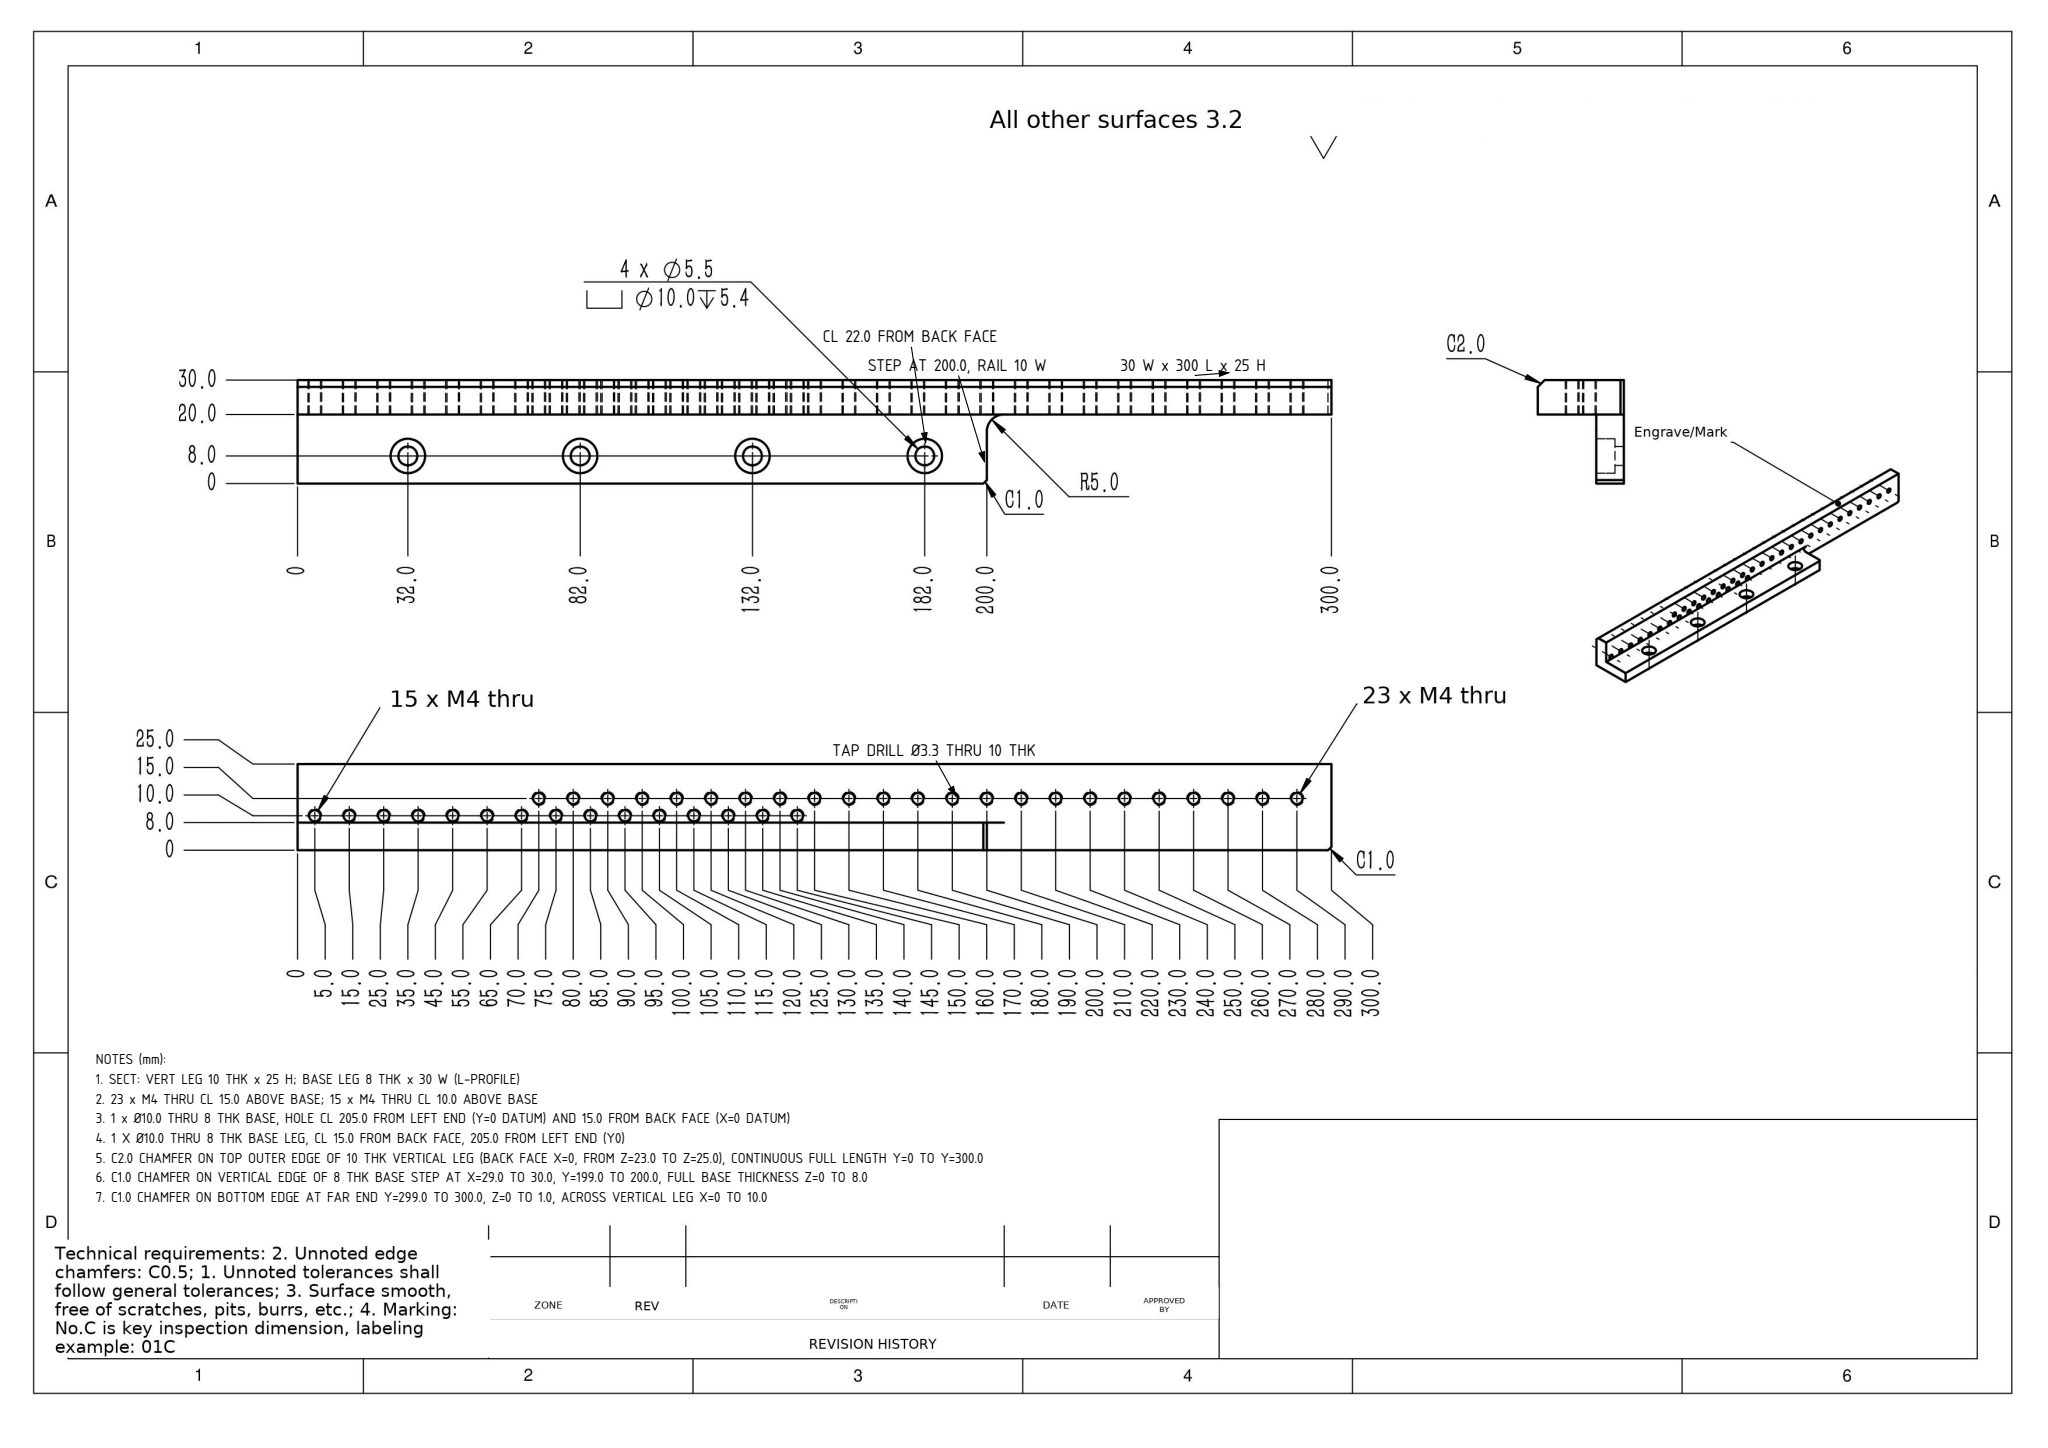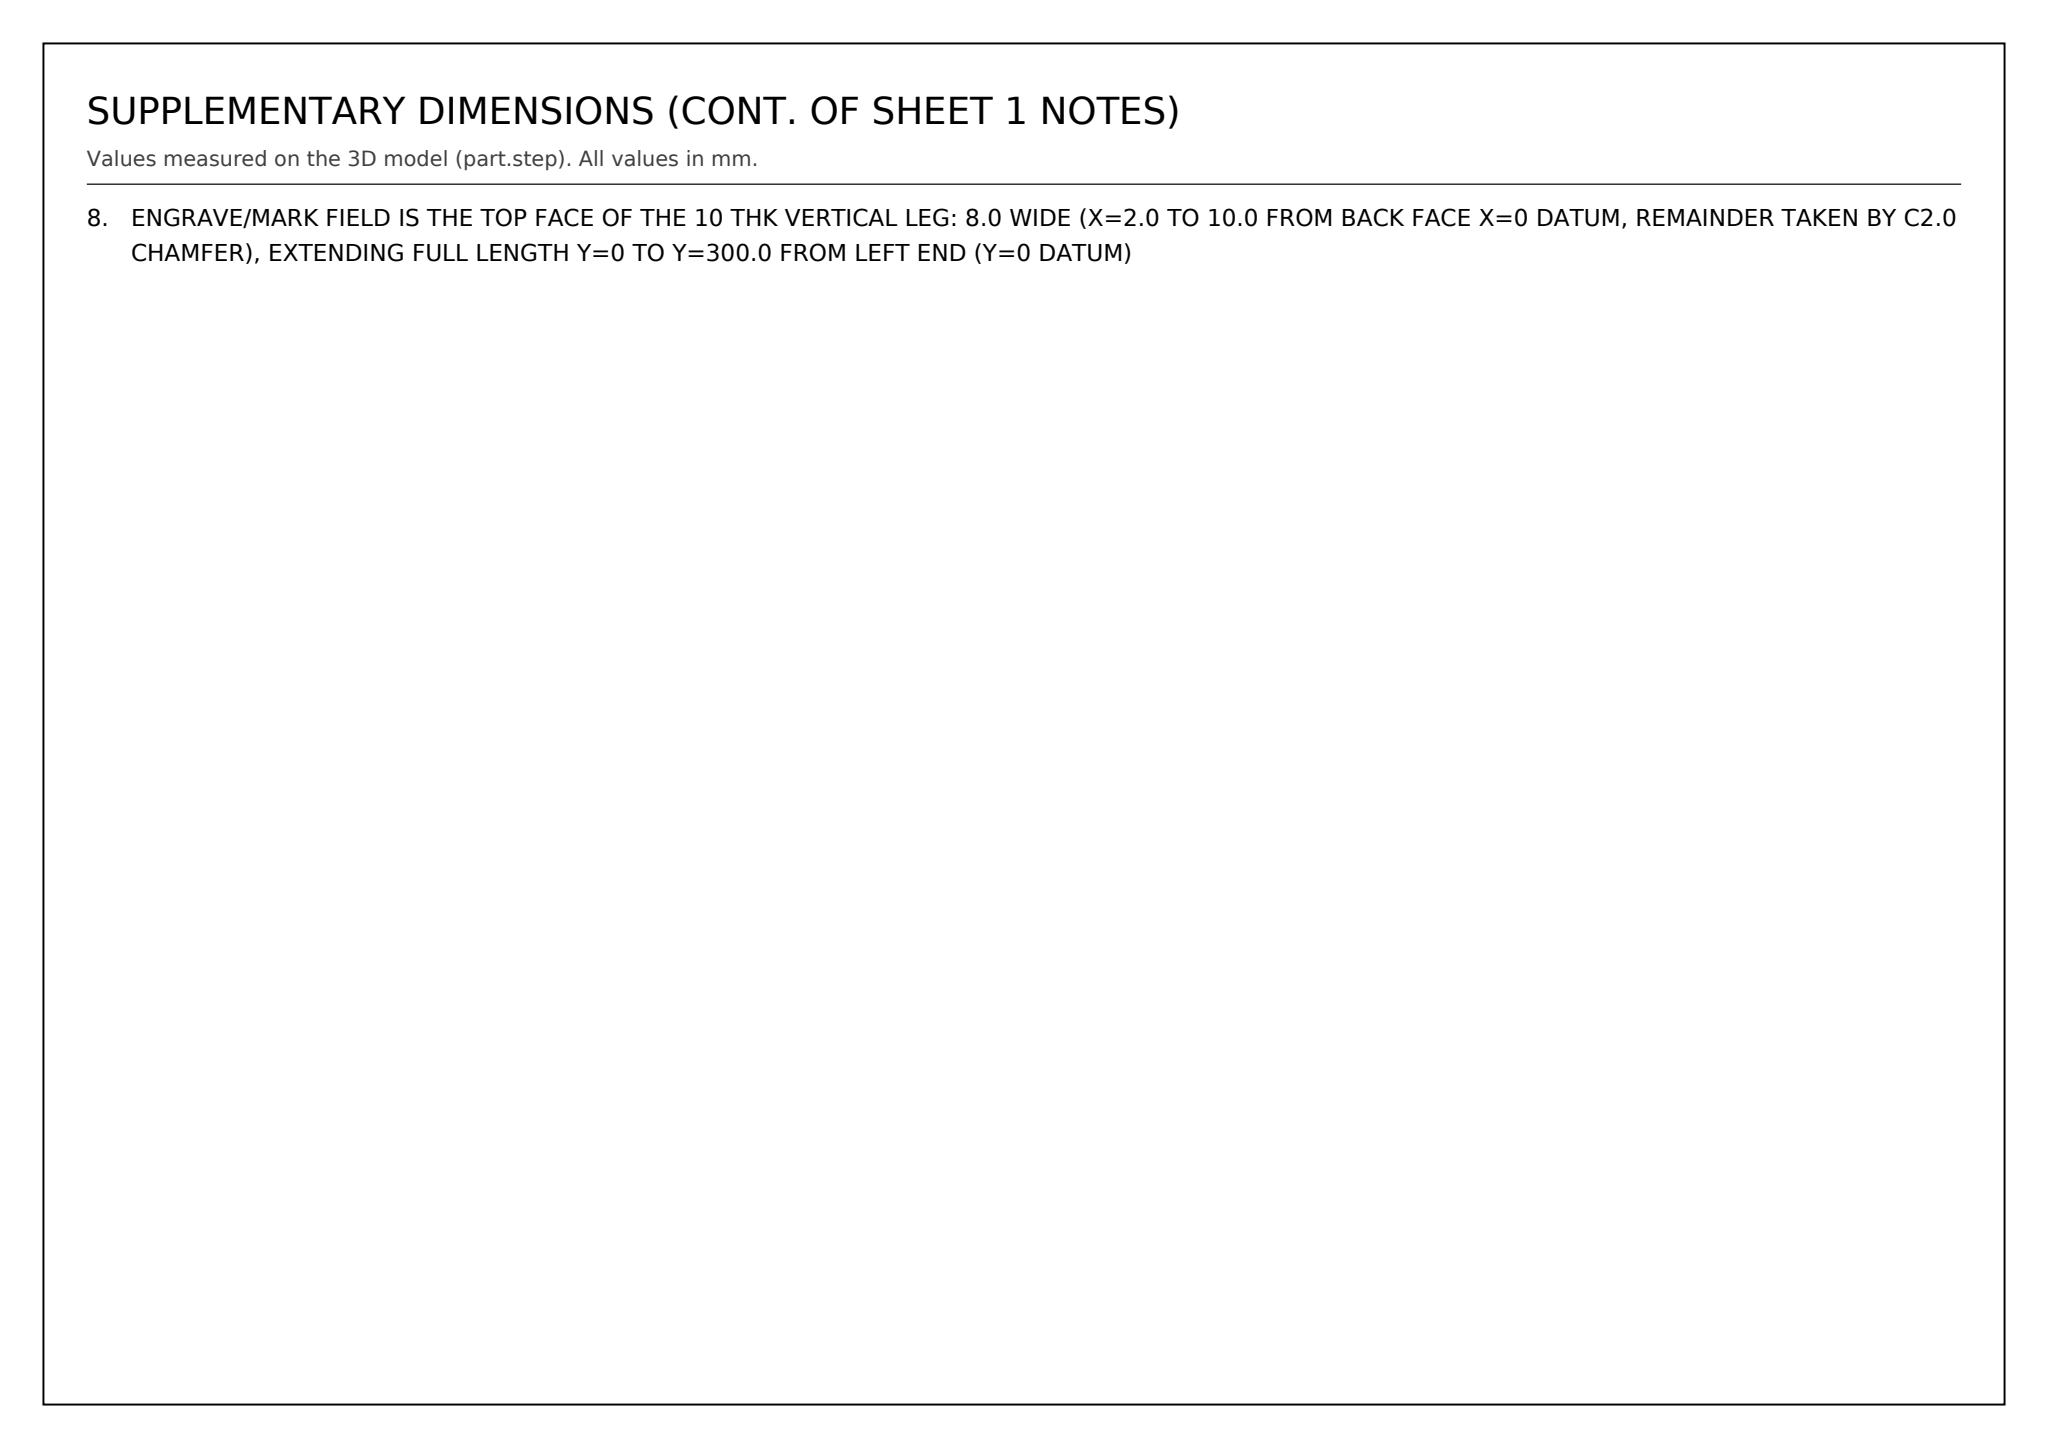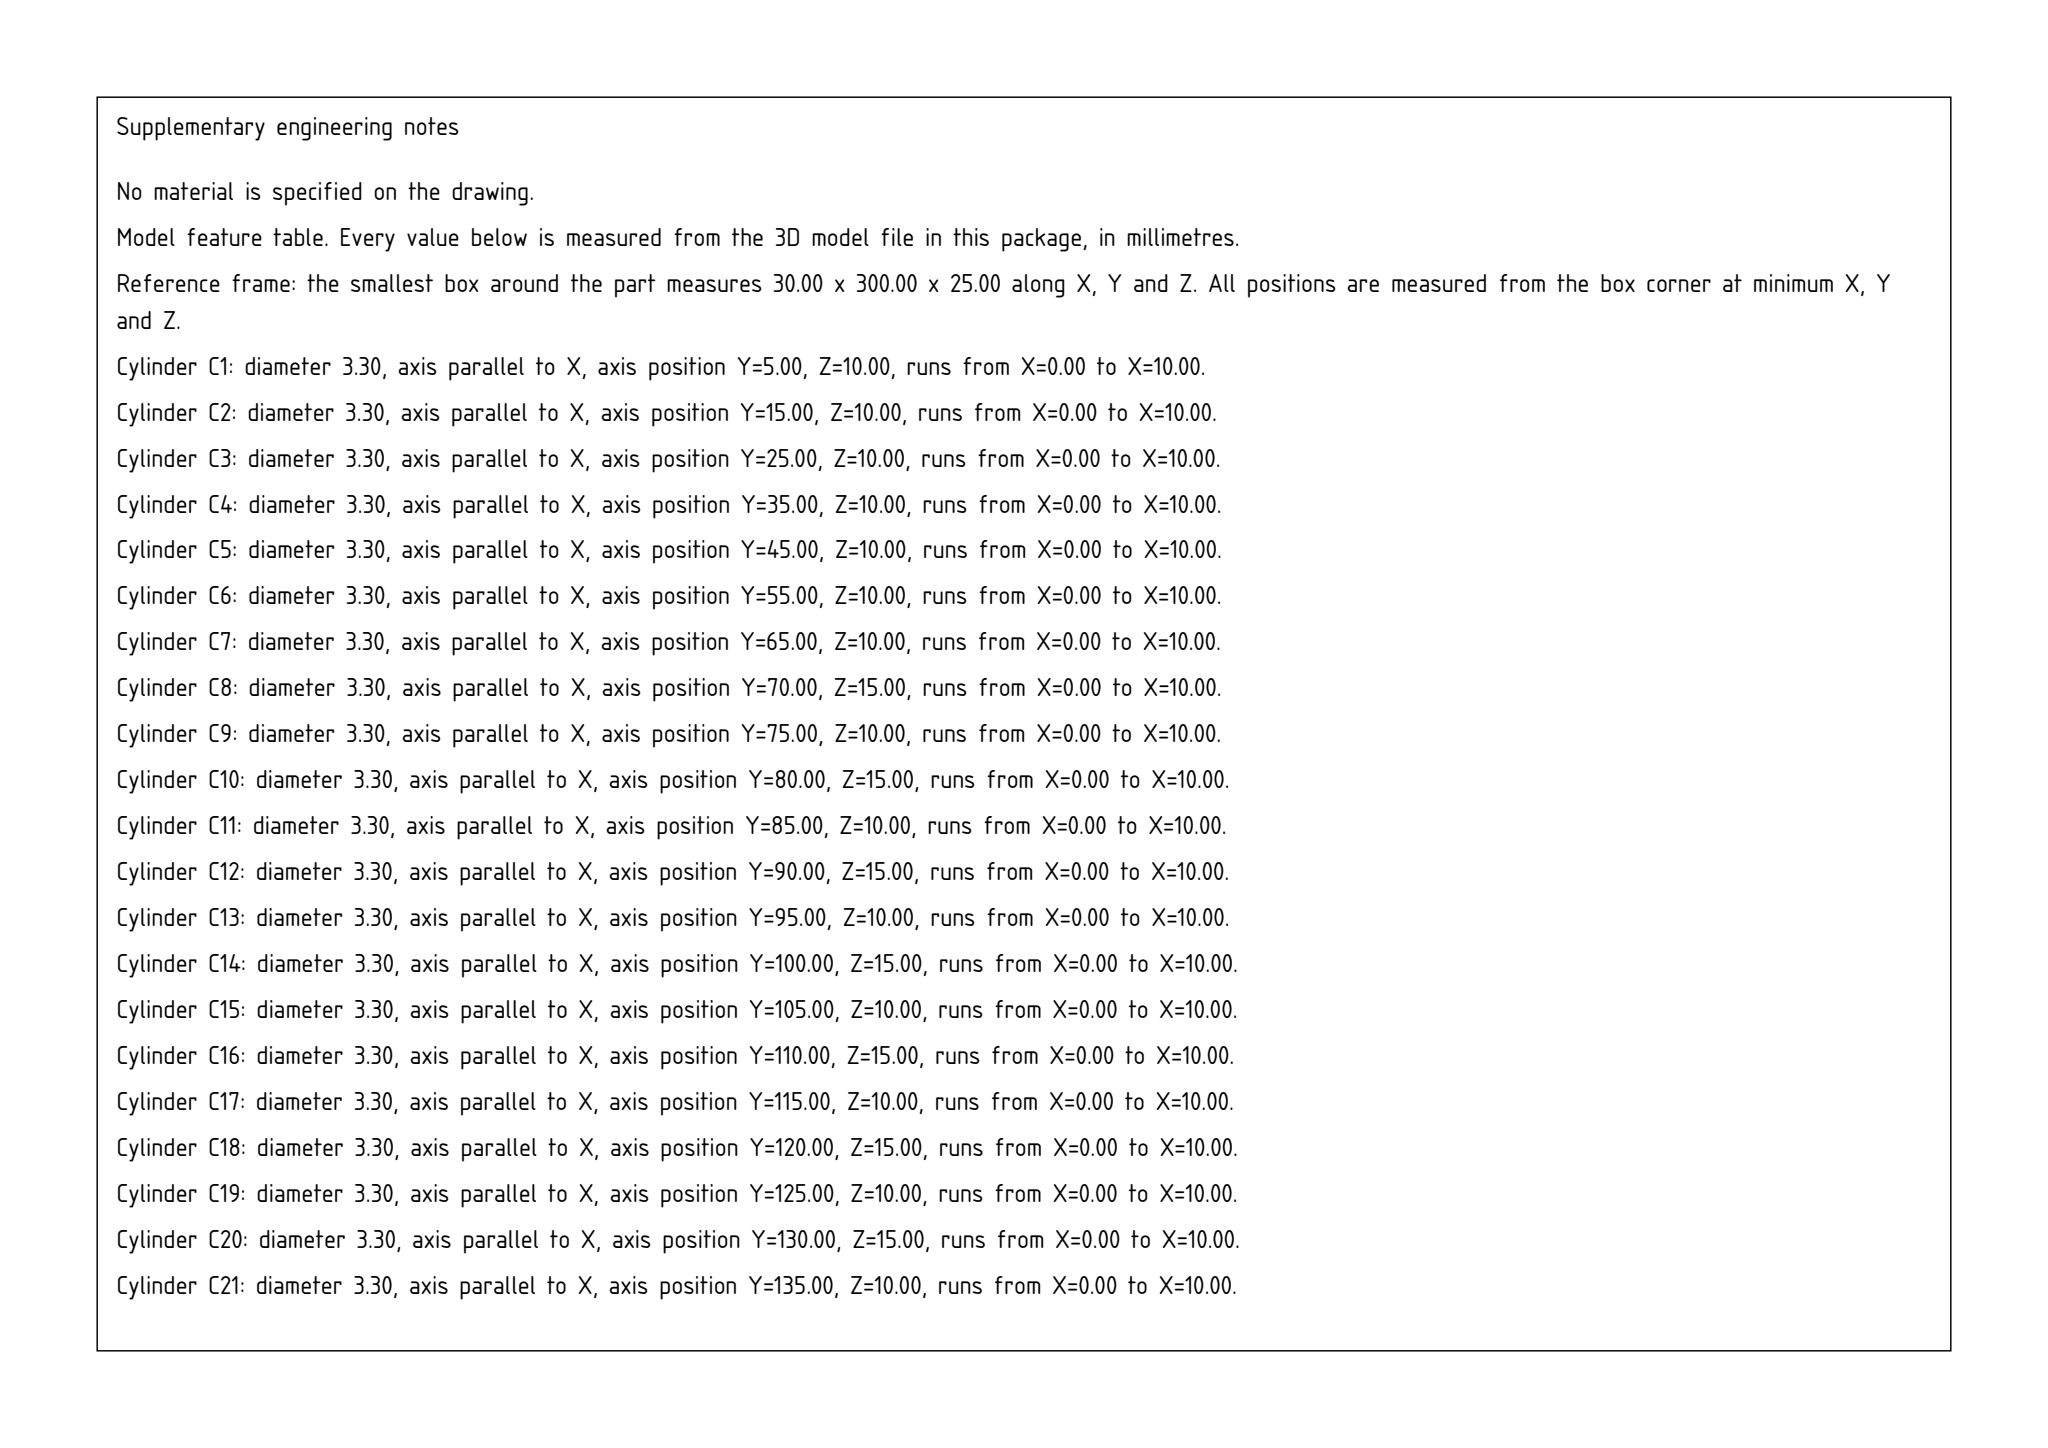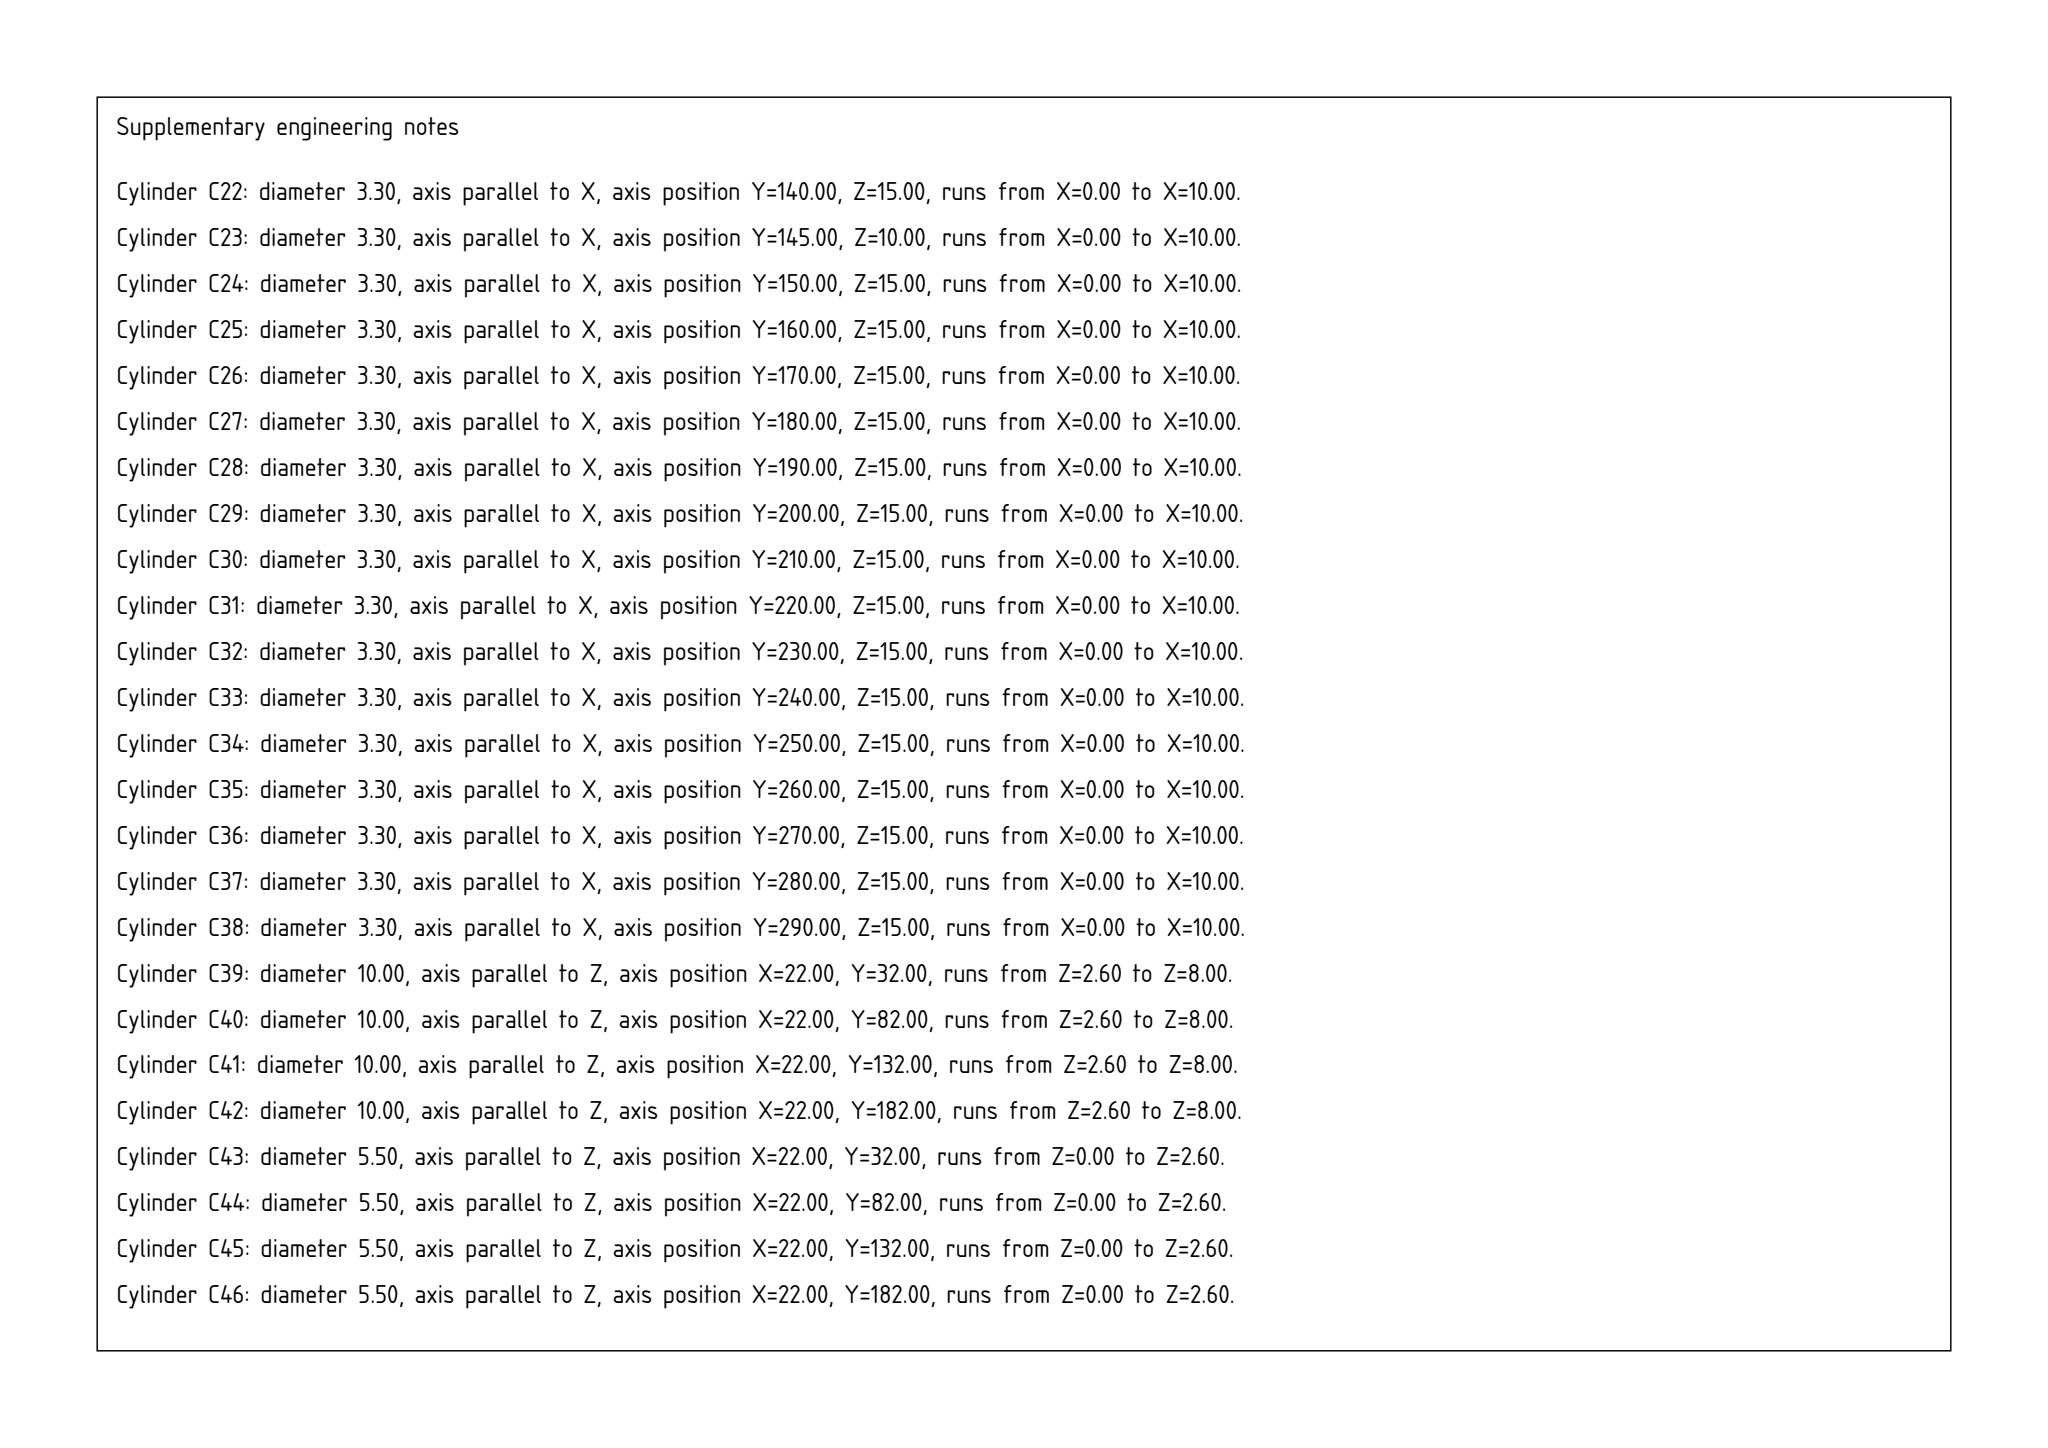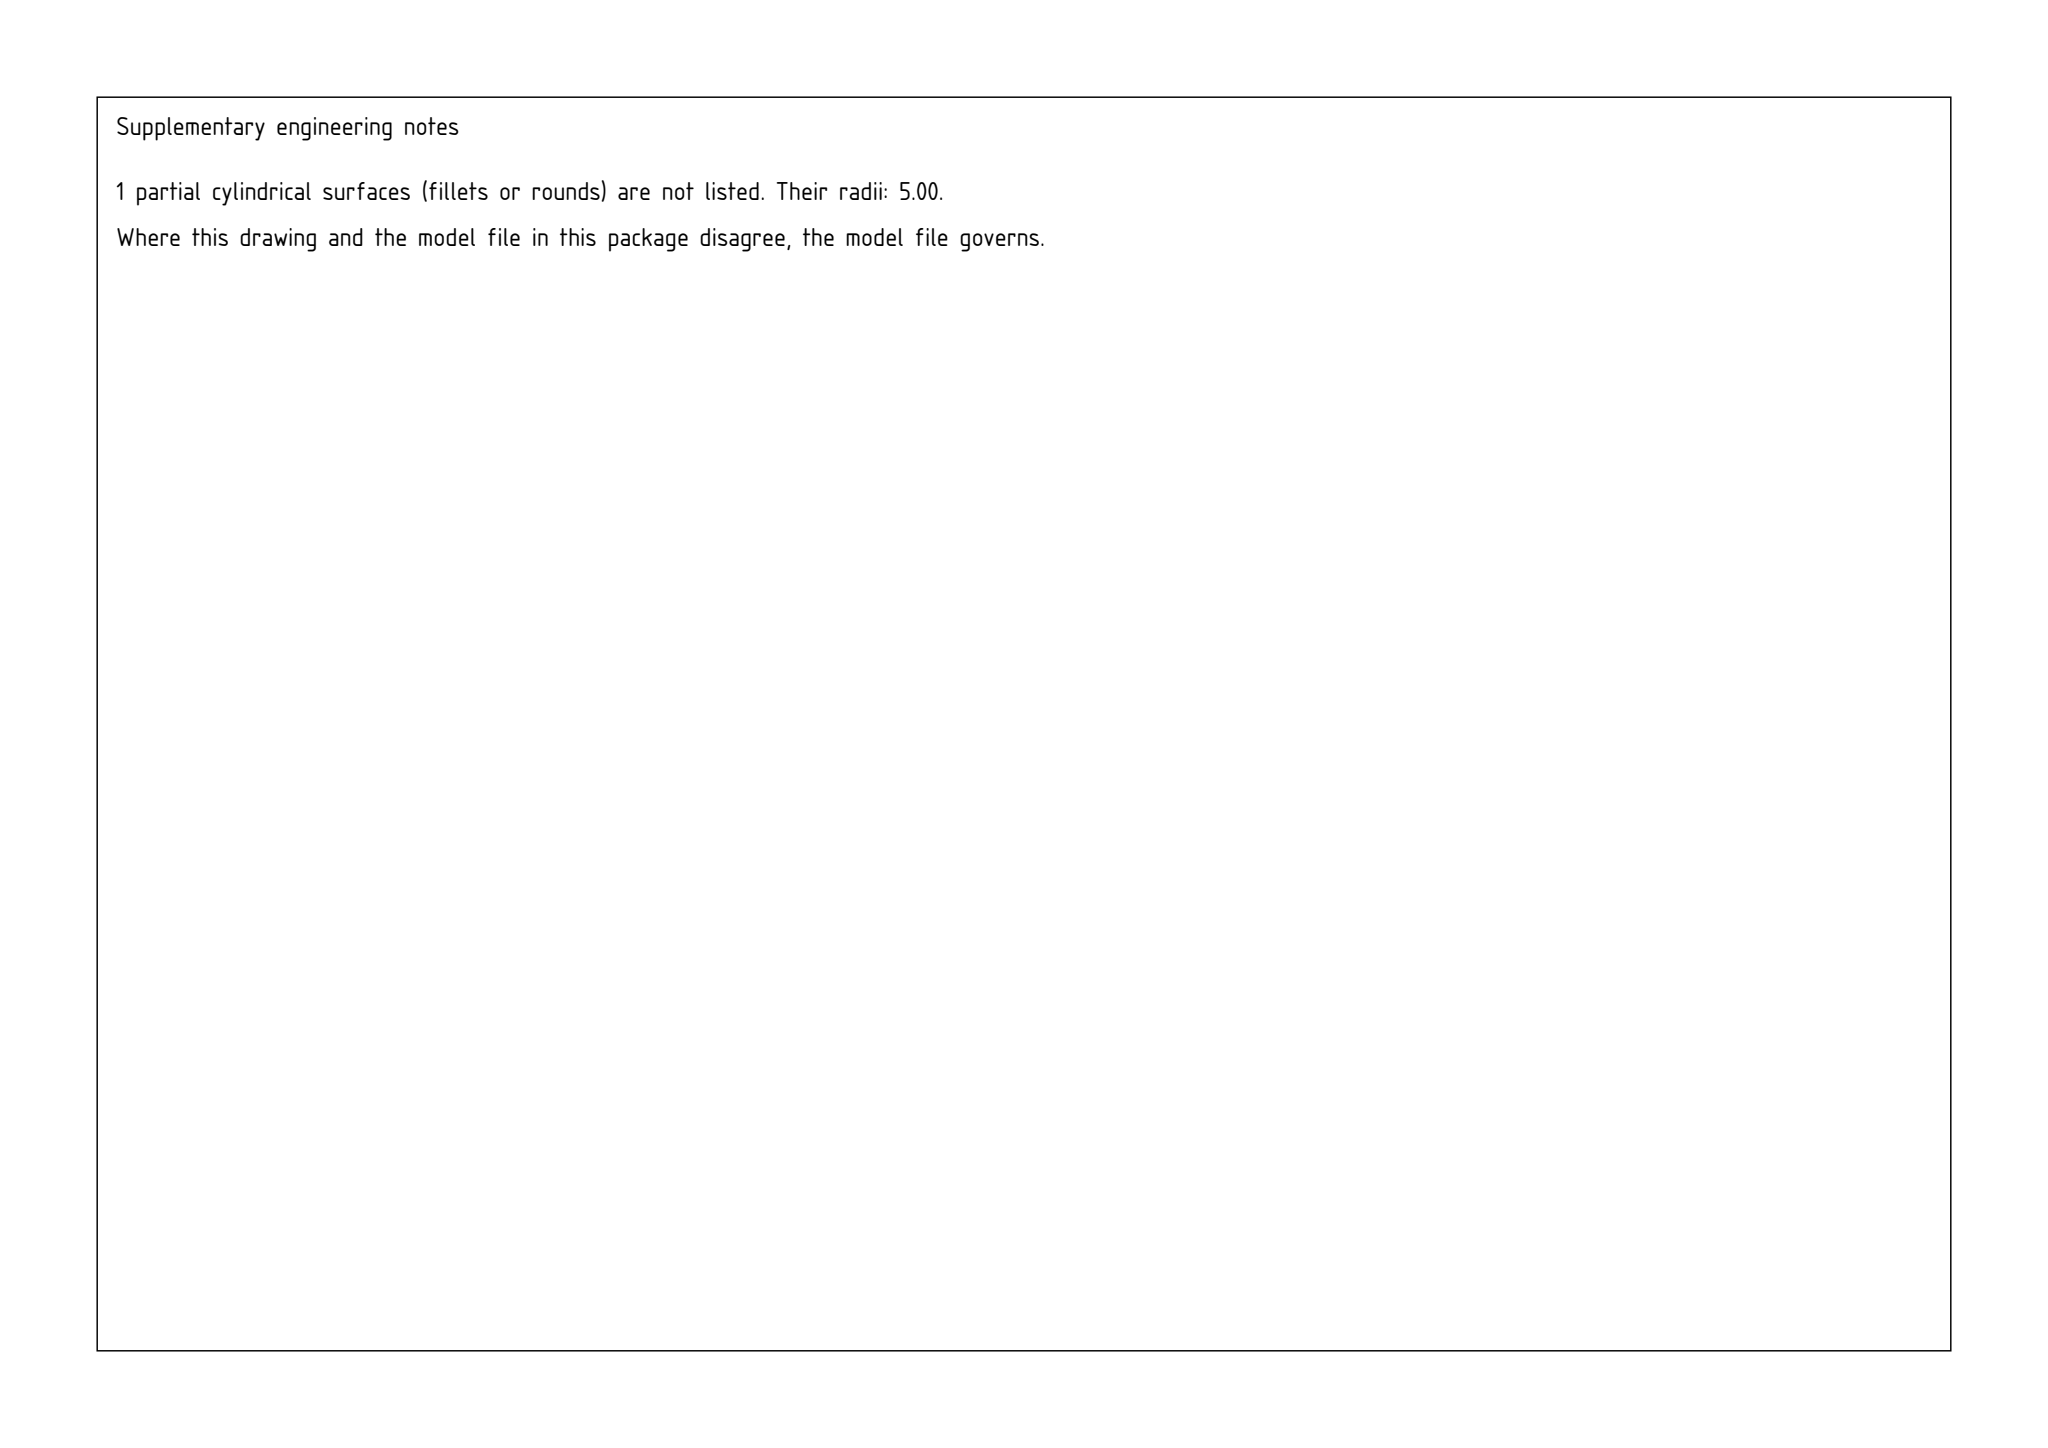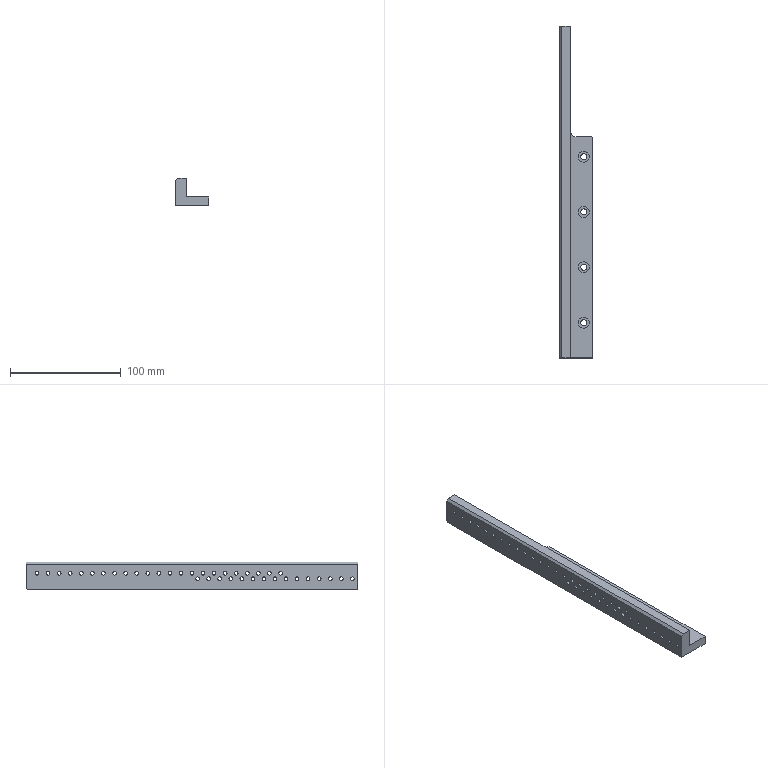Part | SolidWorks | mm | 1 solid | 109 faces | box 30 x 300 x 25 mm | volume 101240 mm3 | cylinder 93 | plane 16 | commonest cylinder face diameters 3.3 x76 10 x9 5.5 x8
Drawing notes:
OA SIZE 30 W x 300 L x 25 H | from the solid: bbox_xyz 30.0 x 300.0 x 25.0
SECT: VERT LEG 10 THK x 25 H; BASE LEG 8 THK x 30 W (L-PROFILE) | from the solid: planes x=0/10/30, z=0/8/25; bbox 30 x 300 x 25
STEP AT 200.0: BASE 30 W x 8 THK ENDS, R5.0; 10 W RAIL CONT TO 300 | from the solid: plane y=200 ends base leg; wall x=0-10 runs to y=300; R5.0 callout
23 x M4 THRU CL 15.0 ABOVE BASE; 15 x M4 THRU CL 10.0 ABOVE BASE | from the solid: Ø3.3 x-axis holes L=10 thru wall at z=15 (23 off) and z=10 (15 off)
4 x Ø5.5 THRU 8 THK BASE, CL 22.0 FROM BACK FACE; CBORE Ø10 DP 5.4 FROM TOP | from the solid: Ø5.5 L=2.6 and Ø10 L=5.4 z-axis holes at x=22.0, y=32/82/132/182
1 x Ø10.0 THRU 8 THK BASE, HOLE CL 205.0 FROM LEFT END (Y=0 DATUM) AND 15.0 FROM BACK FACE (X=0 DATUM) | from the solid: cylinders: [10.0,"z",[15.0,205.0,null],8.0,1] with base plane z 0.0 to 8.0
ALL M4 THRU HOLES: TAP DRILL Ø3.3, THRU 10.0 THK VERTICAL LEG (X=0 TO X=10.0), AXES PARALLEL TO X | from the solid: cylinders: 3.3 dia, axis x, length 10.0, at z=10.0 and z=15.0; planes x 0.0 and x 10.0
1 X Ø10.0 THRU 8 THK BASE LEG, CL 15.0 FROM BACK FACE, 205.0 FROM LEFT END (Y0) | from the solid: cylinder [10.0, axis z, pos (15.0, 205.0), length 8.0, count 1]
C2.0 CHAMFER ON TOP OUTER EDGE OF 10 THK VERTICAL LEG (BACK FACE X=0, FROM Z=23.0 TO Z=25.0), CONTINUOUS FULL LENGTH Y=0 TO Y=300.0 | from the solid: inclined_planes: angle_to_xyz_axes [45,90,45], bbox_from [0.0,0.0,23.0], size [2.0,300.0,2.0]
C1.0 CHAMFER ON VERTICAL EDGE OF 8 THK BASE STEP AT X=29.0 TO 30.0, Y=199.0 TO 200.0, FULL BASE THICKNESS Z=0 TO 8.0 | from the solid: inclined_planes: angle_to_xyz_axes [45,45,90], bbox_from [29.0,199.0,0.0], size [1.0,1.0,8.0]
C1.0 CHAMFER ON BOTTOM EDGE AT FAR END Y=299.0 TO 300.0, Z=0 TO 1.0, ACROSS VERTICAL LEG X=0 TO 10.0 | from the solid: inclined_planes: angle_to_xyz_axes [90,45,45], bbox_from [0.0,299.0,0.0], size [10.0,1.0,1.0]
ENGRAVE/MARK FIELD IS THE TOP FACE OF THE 10 THK VERTICAL LEG: 8.0 WIDE (X=2.0 TO 10.0 FROM BACK FACE X=0 DATUM, REMAINDER TAKEN BY C2.0 CHAMFER), EXTENDING FULL LENGTH Y=0 TO Y=300.0 FROM LEFT END (Y=0 DATUM) | from the solid: axis_planes z=25.0 extent x [2.0,10.0], y [0.0,300.0], area 2400 (top face of vertical leg); inclined_plane 45/90/45 at bbox_from [0,0,23] size [2,300,2] = C2.0 chamfer
build123d program:
from build123d import *

# Parameters (mm, degrees)
SKETCH1_W                                       = 30
SKETCH1_H                                       = 300
BOSS_EXTRUDE1_DEPTH                             = 25
CHAMFER1_SIZE                                   = 2
SKETCH2_W                                       = 20
SKETCH2_H                                       = 300
CUT_EXTRUDE1_DEPTH                              = 17
M4_TAPPED_HOLE1_D                               = 3.3
M5_HEX_SOCKET_HEAD_CAP_SCREW_CBORE1_D           = 5.5
M5_HEX_SOCKET_HEAD_CAP_SCREW_CBORE1_CBORE_D     = 10
M5_HEX_SOCKET_HEAD_CAP_SCREW_CBORE1_CBORE_DEPTH = 5.4
M4_TAPPED_HOLE2_D                               = 3.3
LPATTERN4_COUNT                                 = 6
LPATTERN4_PITCH                                 = 50
LPATTERN5_COUNT                                 = 23
LPATTERN5_PITCH                                 = 10
LPATTERN6_COUNT                                 = 15
LPATTERN6_PITCH                                 = 10
SKETCH9_W                                       = 20
SKETCH9_H                                       = 100
CUT_EXTRUDE2_DEPTH                              = 302.975
FILLET1_R                                       = 5
CHAMFER2_SIZE                                   = 1


with BuildPart() as part:
    # Sketch1 → Boss-Extrude1 (new body)
    with BuildSketch(Plane.XY):
        with Locations((15, 150)):
            Rectangle(SKETCH1_W, SKETCH1_H)
    extrude(amount=BOSS_EXTRUDE1_DEPTH)

    # Chamfer1
    chamfer1_edges = [part.edges().sort_by_distance(p)[0] for p in [
        (0, 150, 25),
    ]]
    chamfer(chamfer1_edges, length=CHAMFER1_SIZE)

    # Sketch2 → Cut-Extrude1 (cut)
    with BuildSketch(Plane.XY.offset(25)):
        with Locations((20, 150)):
            Rectangle(SKETCH2_W, SKETCH2_H)
    extrude(amount=-CUT_EXTRUDE1_DEPTH, mode=Mode.SUBTRACT)

    # M4 Tapped Hole1 (through all)
    with Locations(Plane.ZY):
        with Locations((10, 5)):
            m4_tapped_hole1 = Hole(M4_TAPPED_HOLE1_D / 2)

    # M5 Hex Socket Head Cap Screw CBORE1 (through all)
    with Locations(Plane.XY.offset(8)):
        with Locations((22, 282)):
            m5_hex_socket_head_cap_screw_cbore1 = CounterBoreHole(M5_HEX_SOCKET_HEAD_CAP_SCREW_CBORE1_D / 2, M5_HEX_SOCKET_HEAD_CAP_SCREW_CBORE1_CBORE_D / 2, M5_HEX_SOCKET_HEAD_CAP_SCREW_CBORE1_CBORE_DEPTH)

    # M4 Tapped Hole2 (through all)
    with Locations(Plane.ZY):
        with Locations((15, 290)):
            m4_tapped_hole2 = Hole(M4_TAPPED_HOLE2_D / 2)

    # LPattern4: M5 Hex Socket Head Cap Screw CBORE1 ×6
    with Locations(*[(0, -i * LPATTERN4_PITCH, 0) for i in range(1, LPATTERN4_COUNT)]):
        add(m5_hex_socket_head_cap_screw_cbore1, mode=Mode.SUBTRACT)

    # LPattern5: M4 Tapped Hole2 ×23
    with Locations(*[(0, -i * LPATTERN5_PITCH, 0) for i in range(1, LPATTERN5_COUNT)]):
        add(m4_tapped_hole2, mode=Mode.SUBTRACT)

    # LPattern6: M4 Tapped Hole1 ×15
    with Locations(*[(0, i * LPATTERN6_PITCH, 0) for i in range(1, LPATTERN6_COUNT)]):
        add(m4_tapped_hole1, mode=Mode.SUBTRACT)

    # Sketch9 → Cut-Extrude2 (cut, through all)
    with BuildSketch(Plane.XY.offset(8)):
        with Locations((20, 250)):
            Rectangle(SKETCH9_W, SKETCH9_H)
    extrude(amount=-CUT_EXTRUDE2_DEPTH, mode=Mode.SUBTRACT)

    # Fillet1
    fillet1_edges = [part.edges().sort_by_distance(p)[0] for p in [
        (10, 200, 4),
    ]]
    fillet(fillet1_edges, radius=FILLET1_R)

    # Chamfer2
    chamfer2_edges = [part.edges().sort_by_distance(p)[0] for p in [
        (5, 300, 0),
        (30, 200, 4),
    ]]
    chamfer(chamfer2_edges, length=CHAMFER2_SIZE)


solid = part.part